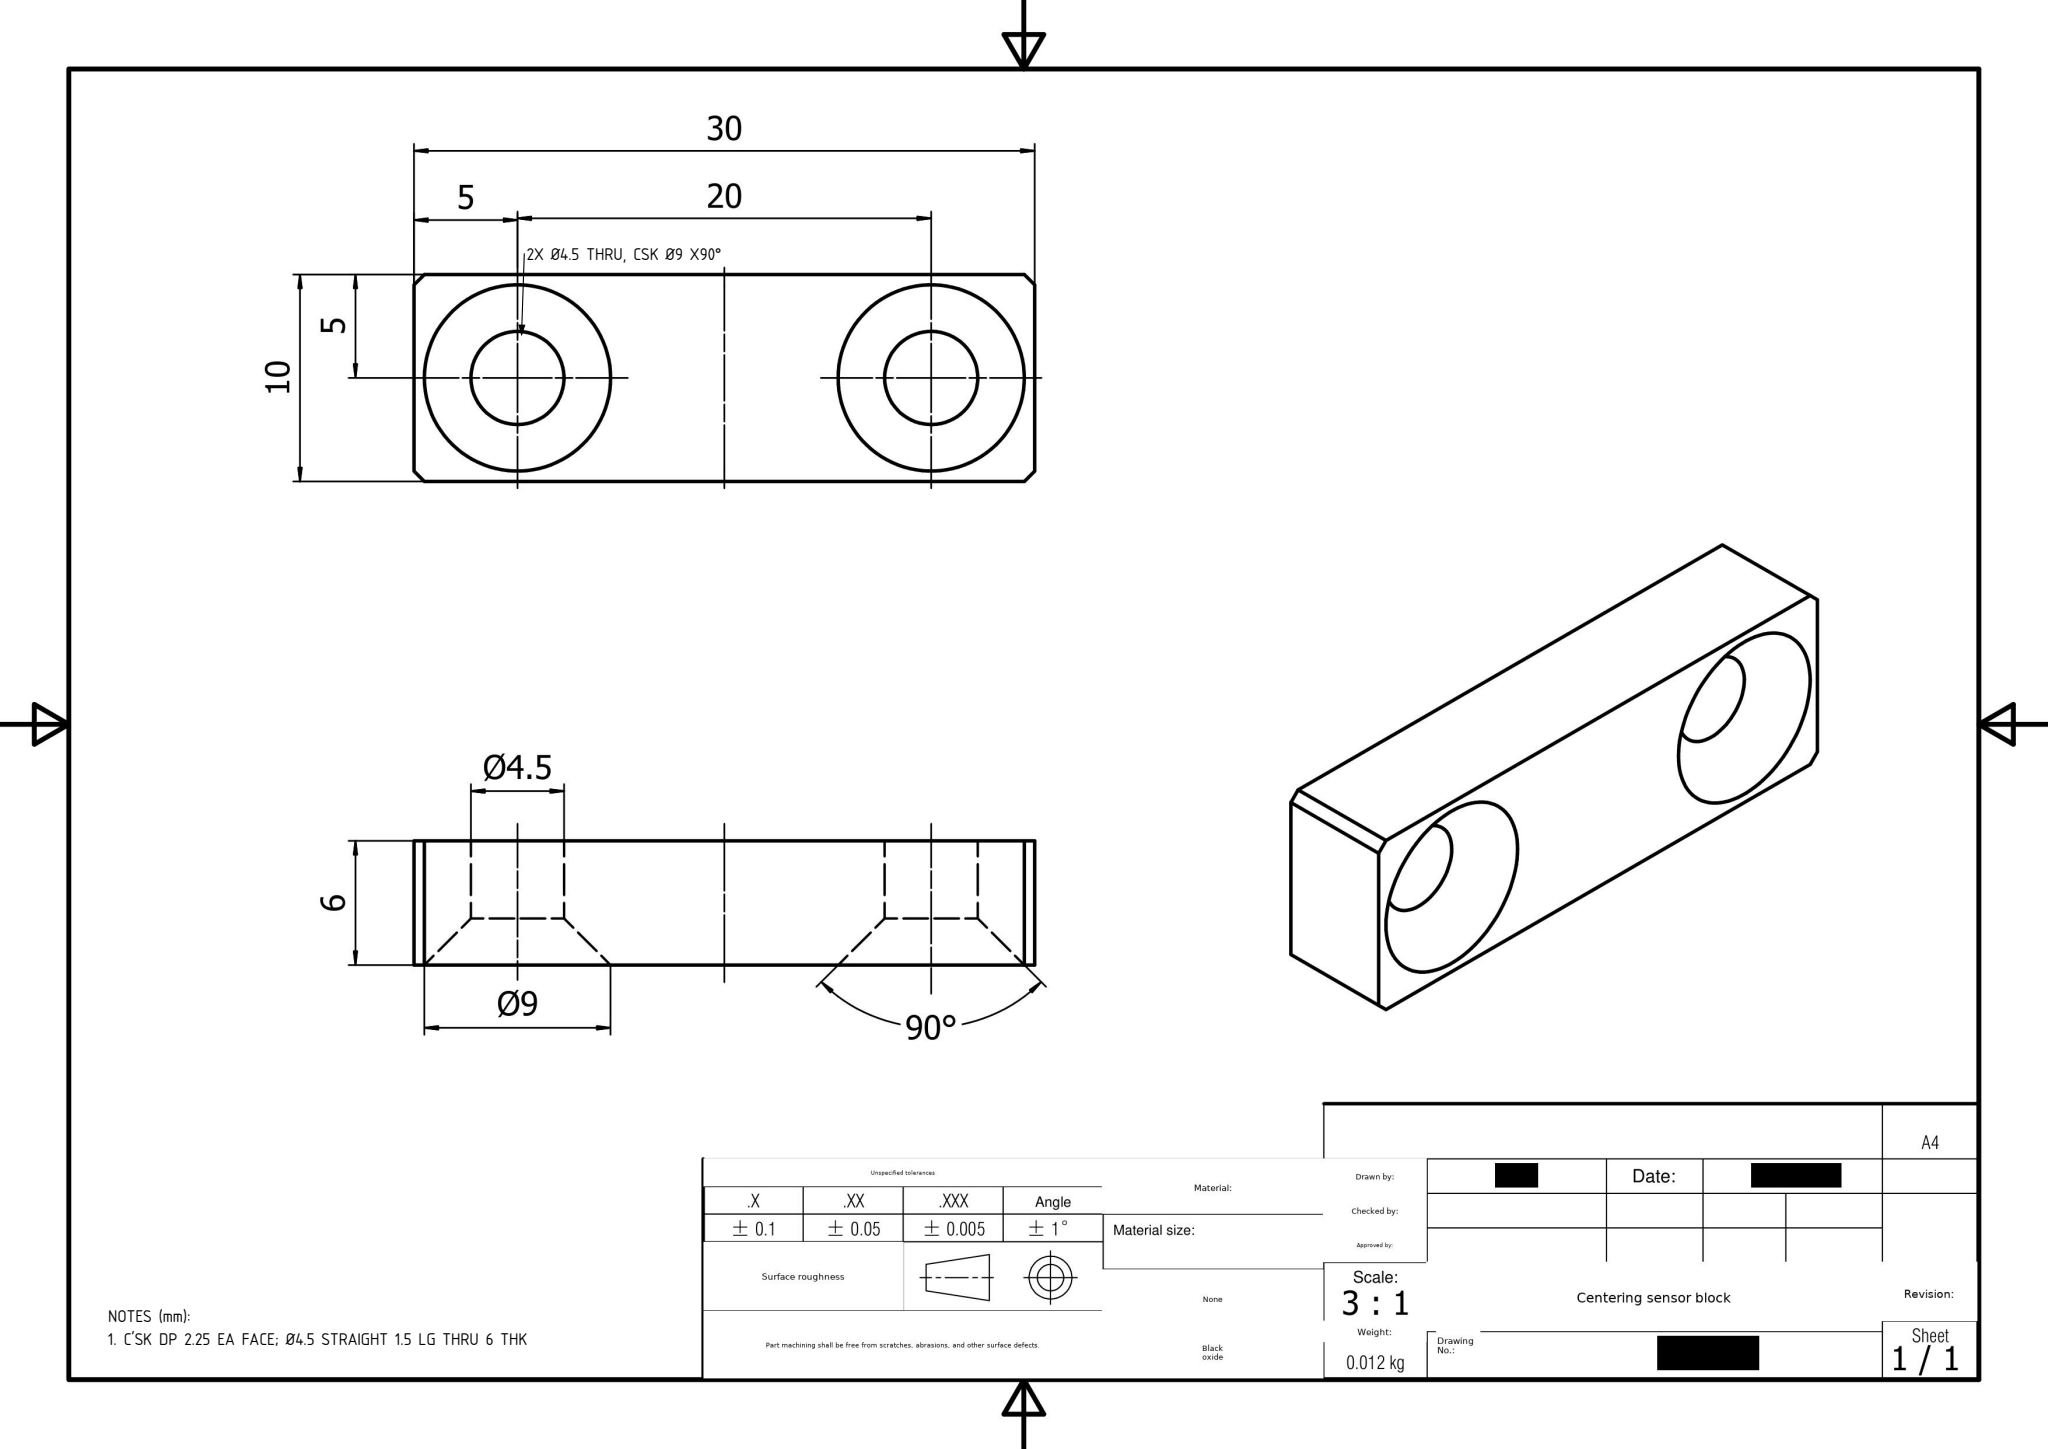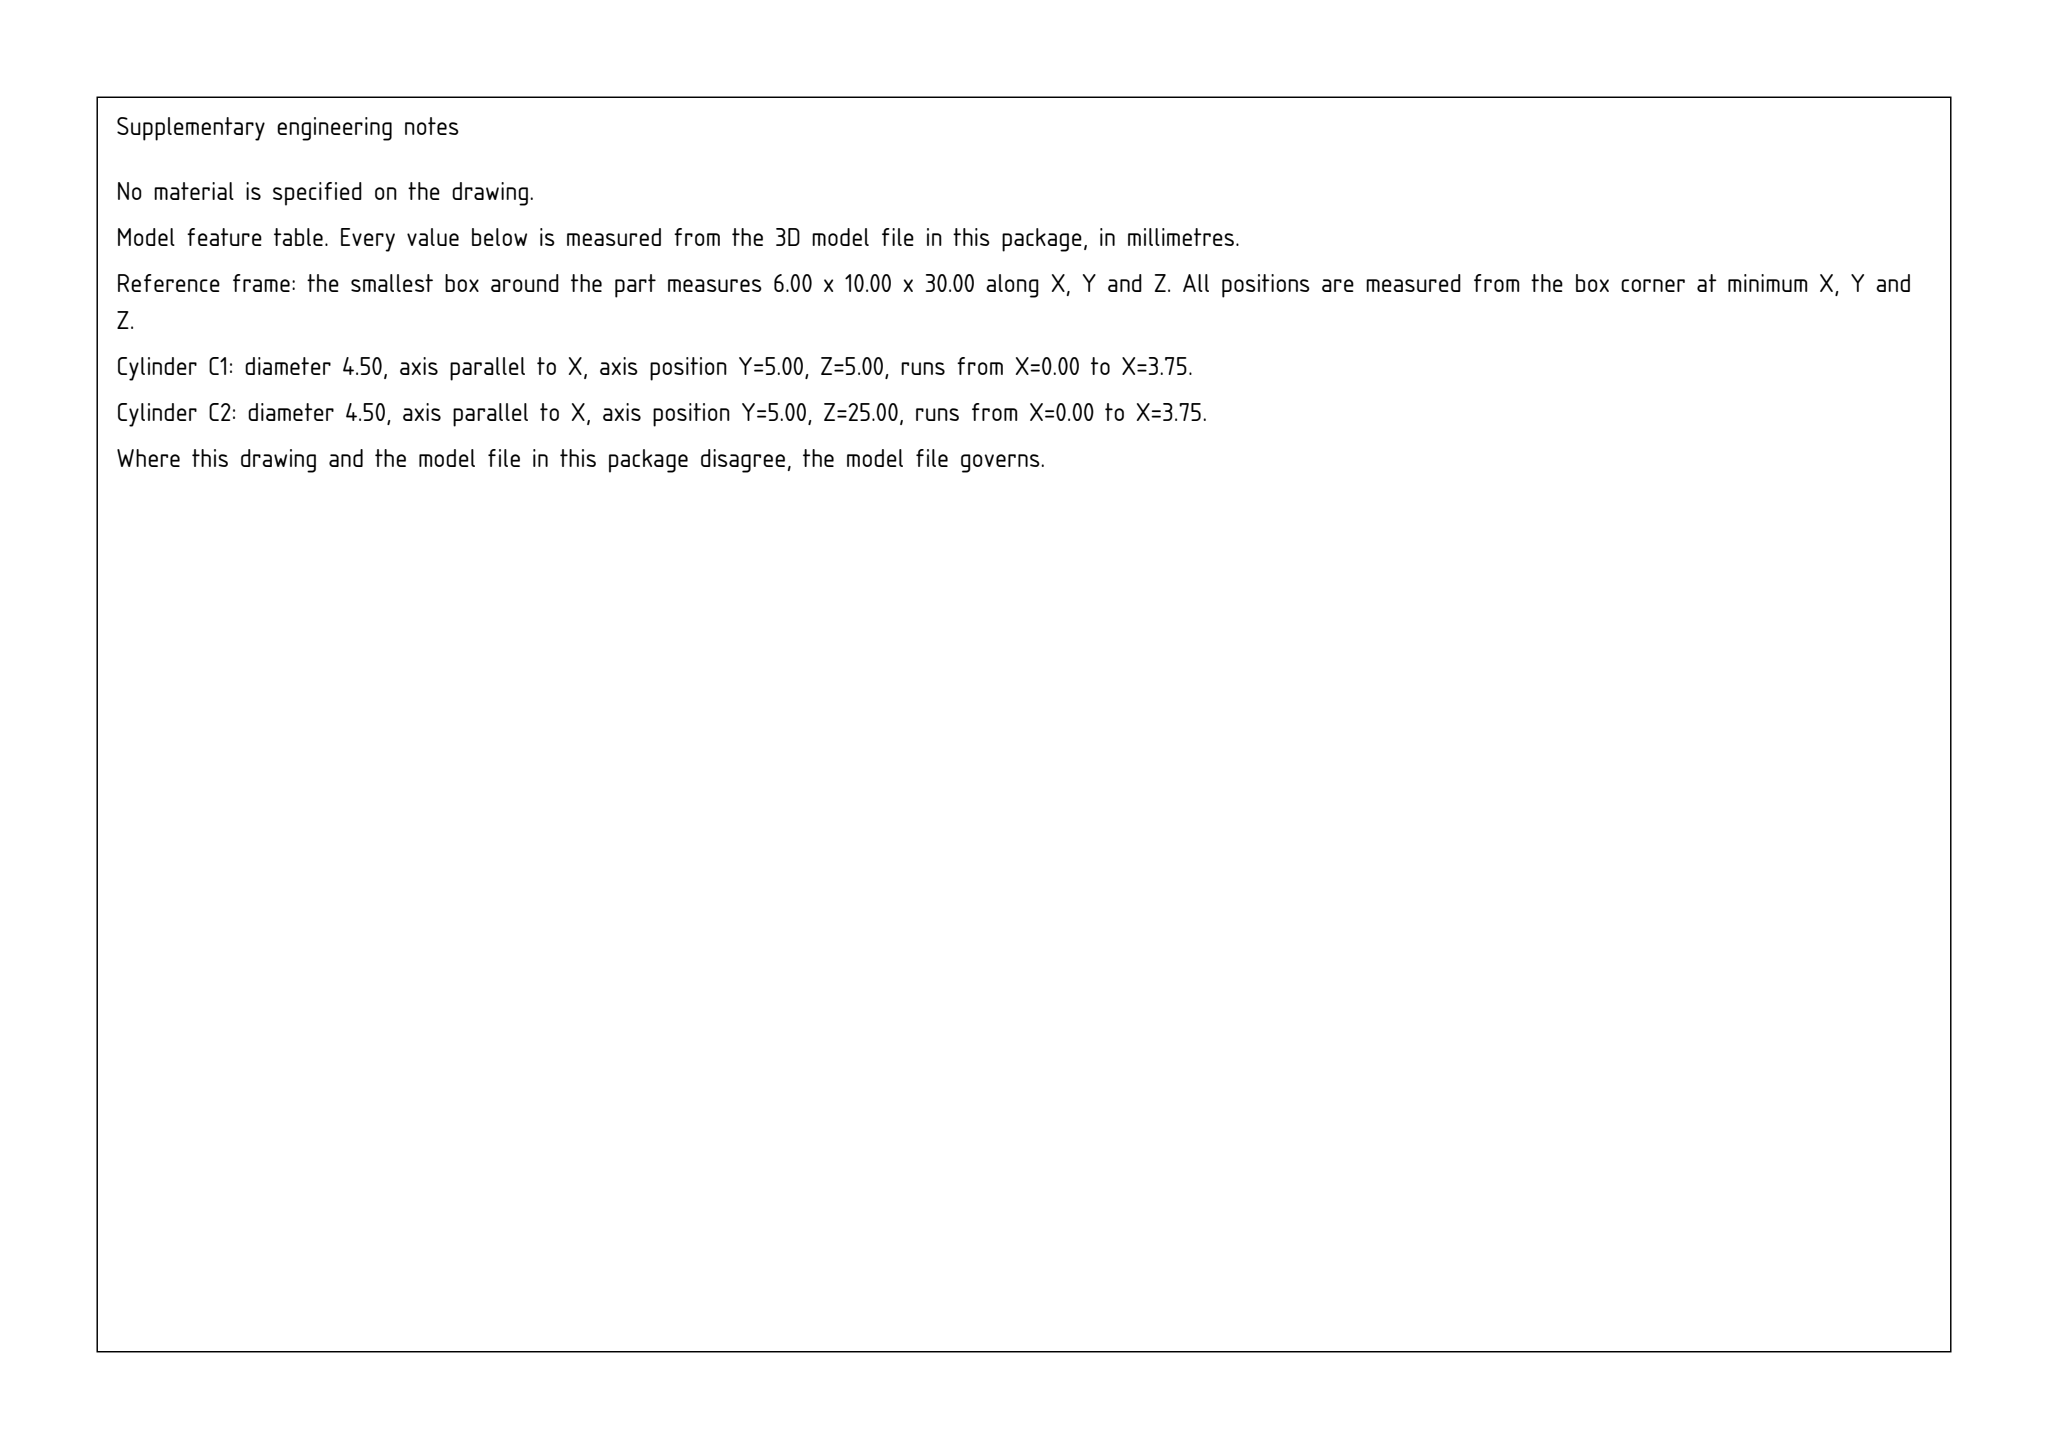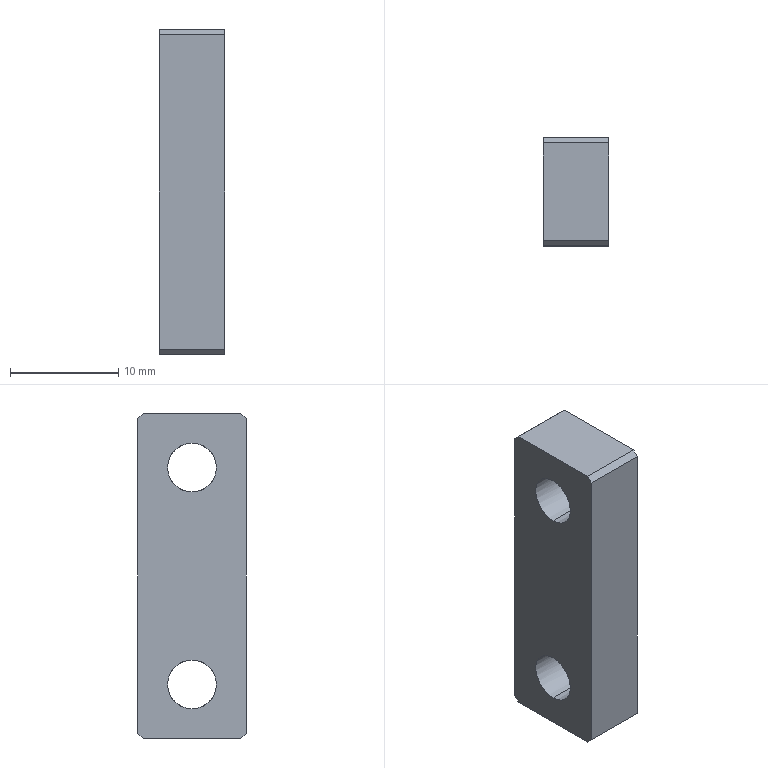Part | SolidWorks | mm | 1 solid | 18 faces | box 6 x 10 x 30 mm | volume 1511 mm3 | plane 10 | cylinder 4 | cone 4 | commonest cylinder face diameters 4.5 x4
Drawing notes:
Ø4.5 THRU, C'SK Ø9 X 90° BOTH FACES - 2 HOLES | from the solid: cylinders Ø4.5 axis x at (y5,z5)&(y5,z25), 2 per hole x 3.75 lg thru 6 thk; cones[90°,ref Ø9] qty 4 = 2 per hole
C'SK DP 2.25 EA FACE; Ø4.5 STRAIGHT 1.5 LG THRU 6 THK | from the solid: (9-4.5)/2=2.25 cone depth per face; bbox x=6, planes x=0 & x=6; 6-2(2.25)=1.5
STEP:
#1=CARTESIAN_POINT('',(0.,0.,-12.25));
#2=VERTEX_POINT('',#1);
#3=CARTESIAN_POINT('',(0.,0.,-7.75));
#4=VERTEX_POINT('',#3);
#5=CARTESIAN_POINT('',(0.,0.,-10.));
#6=DIRECTION('',(-1.,0.,0.));
#7=DIRECTION('',(0.,0.,-1.));
#8=AXIS2_PLACEMENT_3D('',#5,#6,#7);
#9=CIRCLE('',#8,2.25);
#10=EDGE_CURVE('',#2,#4,#9,.T.);
#11=ORIENTED_EDGE('',*,*,#10,.T.);
#12=CARTESIAN_POINT('',(3.75,0.,-7.75));
#13=VERTEX_POINT('',#12);
#14=CARTESIAN_POINT('',(-26.187,0.,-7.75));
#15=DIRECTION('',(1.,0.,0.));
#16=VECTOR('',#15,1000.);
#17=LINE('',#14,#16);
#18=EDGE_CURVE('',#4,#13,#17,.T.);
#19=ORIENTED_EDGE('',*,*,#18,.T.);
#20=CARTESIAN_POINT('',(3.75,-2.25,-10.));
#21=VERTEX_POINT('',#20);
#22=CARTESIAN_POINT('',(3.75,0.,-10.));
#23=DIRECTION('',(-1.,0.,0.));
#24=DIRECTION('',(0.,0.,-1.));
#25=AXIS2_PLACEMENT_3D('',#22,#23,#24);
#26=CIRCLE('',#25,2.25);
#27=EDGE_CURVE('',#21,#13,#26,.T.);
#28=ORIENTED_EDGE('',*,*,#27,.F.);
#29=CARTESIAN_POINT('',(3.75,0.,-12.25));
#30=VERTEX_POINT('',#29);
#31=CARTESIAN_POINT('',(3.75,0.,-10.));
#32=DIRECTION('',(-1.,0.,0.));
#33=DIRECTION('',(0.,0.,-1.));
#34=AXIS2_PLACEMENT_3D('',#31,#32,#33);
#35=CIRCLE('',#34,2.25);
#36=EDGE_CURVE('',#30,#21,#35,.T.);
#37=ORIENTED_EDGE('',*,*,#36,.F.);
#38=CARTESIAN_POINT('',(-26.187,0.,-12.25));
#39=DIRECTION('',(1.,0.,0.));
#40=VECTOR('',#39,1000.);
#41=LINE('',#38,#40);
#42=EDGE_CURVE('',#2,#30,#41,.T.);
#43=ORIENTED_EDGE('',*,*,#42,.F.);
#44=EDGE_LOOP('',(#11,#19,#28,#37,#43));
#45=FACE_OUTER_BOUND('',#44,.T.);
#46=CARTESIAN_POINT('',(-26.187,0.,-10.));
#47=DIRECTION('',(1.,0.,0.));
#48=DIRECTION('',(0.,0.,-1.));
#49=AXIS2_PLACEMENT_3D('',#46,#47,#48);
#50=CYLINDRICAL_SURFACE('',#49,2.25);
#51=ADVANCED_FACE('',(#45),#50,.F.);
#52=CARTESIAN_POINT('',(0.,0.,7.75));
#53=VERTEX_POINT('',#52);
#54=CARTESIAN_POINT('',(0.,0.,12.25));
#55=VERTEX_POINT('',#54);
#56=CARTESIAN_POINT('',(0.,0.,10.));
#57=DIRECTION('',(-1.,0.,0.));
#58=DIRECTION('',(0.,0.,-1.));
#59=AXIS2_PLACEMENT_3D('',#56,#57,#58);
#60=CIRCLE('',#59,2.25);
#61=EDGE_CURVE('',#53,#55,#60,.T.);
#62=ORIENTED_EDGE('',*,*,#61,.T.);
#63=CARTESIAN_POINT('',(3.75,0.,12.25));
#64=VERTEX_POINT('',#63);
#65=CARTESIAN_POINT('',(-26.187,0.,12.25));
#66=DIRECTION('',(1.,0.,0.));
#67=VECTOR('',#66,1000.);
#68=LINE('',#65,#67);
#69=EDGE_CURVE('',#55,#64,#68,.T.);
#70=ORIENTED_EDGE('',*,*,#69,.T.);
#71=CARTESIAN_POINT('',(3.75,-2.25,10.));
#72=VERTEX_POINT('',#71);
#73=CARTESIAN_POINT('',(3.75,0.,10.));
#74=DIRECTION('',(-1.,0.,0.));
#75=DIRECTION('',(0.,0.,-1.));
#76=AXIS2_PLACEMENT_3D('',#73,#74,#75);
#77=CIRCLE('',#76,2.25);
#78=EDGE_CURVE('',#72,#64,#77,.T.);
#79=ORIENTED_EDGE('',*,*,#78,.F.);
#80=CARTESIAN_POINT('',(3.75,0.,7.75));
#81=VERTEX_POINT('',#80);
#82=CARTESIAN_POINT('',(3.75,0.,10.));
#83=DIRECTION('',(-1.,0.,0.));
#84=DIRECTION('',(0.,0.,-1.));
#85=AXIS2_PLACEMENT_3D('',#82,#83,#84);
#86=CIRCLE('',#85,2.25);
#87=EDGE_CURVE('',#81,#72,#86,.T.);
#88=ORIENTED_EDGE('',*,*,#87,.F.);
#89=CARTESIAN_POINT('',(-26.187,0.,7.75));
#90=DIRECTION('',(1.,0.,0.));
#91=VECTOR('',#90,1000.);
#92=LINE('',#89,#91);
#93=EDGE_CURVE('',#53,#81,#92,.T.);
#94=ORIENTED_EDGE('',*,*,#93,.F.);
#95=EDGE_LOOP('',(#62,#70,#79,#88,#94));
#96=FACE_OUTER_BOUND('',#95,.T.);
#97=CARTESIAN_POINT('',(-26.187,0.,10.));
#98=DIRECTION('',(1.,0.,0.));
#99=DIRECTION('',(0.,0.,-1.));
#100=AXIS2_PLACEMENT_3D('',#97,#98,#99);
#101=CYLINDRICAL_SURFACE('',#100,2.25);
#102=ADVANCED_FACE('',(#96),#101,.F.);
#103=CARTESIAN_POINT('',(3.75,2.25,-10.));
#104=VERTEX_POINT('',#103);
#105=CARTESIAN_POINT('',(3.75,0.,-10.));
#106=DIRECTION('',(-1.,0.,0.));
#107=DIRECTION('',(0.,0.,-1.));
#108=AXIS2_PLACEMENT_3D('',#105,#106,#107);
#109=CIRCLE('',#108,2.25);
#110=EDGE_CURVE('',#104,#30,#109,.T.);
#111=ORIENTED_EDGE('',*,*,#110,.T.);
#112=ORIENTED_EDGE('',*,*,#36,.T.);
#113=CARTESIAN_POINT('',(6.,-4.5,-10.));
#114=VERTEX_POINT('',#113);
#115=CARTESIAN_POINT('',(6.,-4.5,-10.));
#116=DIRECTION('',(0.7071,-0.7071,0.));
#117=VECTOR('',#116,1000.);
#118=LINE('',#115,#117);
#119=EDGE_CURVE('',#21,#114,#118,.T.);
#120=ORIENTED_EDGE('',*,*,#119,.T.);
#121=CARTESIAN_POINT('',(6.,4.5,-10.));
#122=VERTEX_POINT('',#121);
#123=CARTESIAN_POINT('',(6.,0.,-10.));
#124=DIRECTION('',(-1.,-0.,0.));
#125=DIRECTION('',(-0.,1.,0.));
#126=AXIS2_PLACEMENT_3D('',#123,#124,#125);
#127=CIRCLE('',#126,4.5);
#128=EDGE_CURVE('',#122,#114,#127,.T.);
#129=ORIENTED_EDGE('',*,*,#128,.F.);
#130=CARTESIAN_POINT('',(6.,4.5,-10.));
#131=DIRECTION('',(0.7071,0.7071,0.));
#132=VECTOR('',#131,1000.);
#133=LINE('',#130,#132);
#134=EDGE_CURVE('',#104,#122,#133,.T.);
#135=ORIENTED_EDGE('',*,*,#134,.F.);
#136=EDGE_LOOP('',(#111,#112,#120,#129,#135));
#137=FACE_OUTER_BOUND('',#136,.T.);
#138=CARTESIAN_POINT('',(6.,0.,-10.));
#139=DIRECTION('',(1.,0.,0.));
#140=DIRECTION('',(-0.,1.,0.));
#141=AXIS2_PLACEMENT_3D('',#138,#139,#140);
#142=CONICAL_SURFACE('',#141,4.5,0.7854);
#143=ADVANCED_FACE('',(#137),#142,.F.);
#144=CARTESIAN_POINT('',(3.75,2.25,10.));
#145=VERTEX_POINT('',#144);
#146=CARTESIAN_POINT('',(3.75,0.,10.));
#147=DIRECTION('',(-1.,0.,0.));
#148=DIRECTION('',(0.,0.,-1.));
#149=AXIS2_PLACEMENT_3D('',#146,#147,#148);
#150=CIRCLE('',#149,2.25);
#151=EDGE_CURVE('',#145,#81,#150,.T.);
#152=ORIENTED_EDGE('',*,*,#151,.T.);
#153=ORIENTED_EDGE('',*,*,#87,.T.);
#154=CARTESIAN_POINT('',(6.,-4.5,10.));
#155=VERTEX_POINT('',#154);
#156=CARTESIAN_POINT('',(6.,-4.5,10.));
#157=DIRECTION('',(0.7071,-0.7071,0.));
#158=VECTOR('',#157,1000.);
#159=LINE('',#156,#158);
#160=EDGE_CURVE('',#72,#155,#159,.T.);
#161=ORIENTED_EDGE('',*,*,#160,.T.);
#162=CARTESIAN_POINT('',(6.,4.5,10.));
#163=VERTEX_POINT('',#162);
#164=CARTESIAN_POINT('',(6.,0.,10.));
#165=DIRECTION('',(-1.,-0.,0.));
#166=DIRECTION('',(-0.,1.,0.));
#167=AXIS2_PLACEMENT_3D('',#164,#165,#166);
#168=CIRCLE('',#167,4.5);
#169=EDGE_CURVE('',#163,#155,#168,.T.);
#170=ORIENTED_EDGE('',*,*,#169,.F.);
#171=CARTESIAN_POINT('',(6.,4.5,10.));
#172=DIRECTION('',(0.7071,0.7071,0.));
#173=VECTOR('',#172,1000.);
#174=LINE('',#171,#173);
#175=EDGE_CURVE('',#145,#163,#174,.T.);
#176=ORIENTED_EDGE('',*,*,#175,.F.);
#177=EDGE_LOOP('',(#152,#153,#161,#170,#176));
#178=FACE_OUTER_BOUND('',#177,.T.);
#179=CARTESIAN_POINT('',(6.,0.,10.));
#180=DIRECTION('',(1.,0.,0.));
#181=DIRECTION('',(0.,1.,0.));
#182=AXIS2_PLACEMENT_3D('',#179,#180,#181);
#183=CONICAL_SURFACE('',#182,4.5,0.7854);
#184=ADVANCED_FACE('',(#178),#183,.F.);
#185=ORIENTED_EDGE('',*,*,#10,.F.);
#186=CARTESIAN_POINT('',(0.,0.,-10.));
#187=DIRECTION('',(-1.,0.,0.));
#188=DIRECTION('',(0.,0.,-1.));
#189=AXIS2_PLACEMENT_3D('',#186,#187,#188);
#190=CIRCLE('',#189,2.25);
#191=EDGE_CURVE('',#4,#2,#190,.T.);
#192=ORIENTED_EDGE('',*,*,#191,.F.);
#193=EDGE_LOOP('',(#185,#192));
#194=FACE_BOUND('',#193,.T.);
#195=ORIENTED_EDGE('',*,*,#61,.F.);
#196=CARTESIAN_POINT('',(0.,0.,10.));
#197=DIRECTION('',(-1.,0.,0.));
#198=DIRECTION('',(0.,0.,-1.));
#199=AXIS2_PLACEMENT_3D('',#196,#197,#198);
#200=CIRCLE('',#199,2.25);
#201=EDGE_CURVE('',#55,#53,#200,.T.);
#202=ORIENTED_EDGE('',*,*,#201,.F.);
#203=EDGE_LOOP('',(#195,#202));
#204=FACE_BOUND('',#203,.T.);
#205=CARTESIAN_POINT('',(0.,-5.,14.5));
#206=VERTEX_POINT('',#205);
#207=CARTESIAN_POINT('',(0.,-5.,-14.5));
#208=VERTEX_POINT('',#207);
#209=CARTESIAN_POINT('',(0.,-5.,0.));
#210=DIRECTION('',(0.,0.,-1.));
#211=VECTOR('',#210,1000.);
#212=LINE('',#209,#211);
#213=EDGE_CURVE('',#206,#208,#212,.T.);
#214=ORIENTED_EDGE('',*,*,#213,.F.);
#215=CARTESIAN_POINT('',(0.,-4.5,15.));
#216=VERTEX_POINT('',#215);
#217=CARTESIAN_POINT('',(0.,-4.75,14.75));
#218=DIRECTION('',(0.,-0.7071,-0.7071));
#219=VECTOR('',#218,1000.);
#220=LINE('',#217,#219);
#221=EDGE_CURVE('',#216,#206,#220,.T.);
#222=ORIENTED_EDGE('',*,*,#221,.F.);
#223=CARTESIAN_POINT('',(0.,4.5,15.));
#224=VERTEX_POINT('',#223);
#225=CARTESIAN_POINT('',(0.,0.,15.));
#226=DIRECTION('',(0.,-1.,0.));
#227=VECTOR('',#226,1000.);
#228=LINE('',#225,#227);
#229=EDGE_CURVE('',#224,#216,#228,.T.);
#230=ORIENTED_EDGE('',*,*,#229,.F.);
#231=CARTESIAN_POINT('',(0.,5.,14.5));
#232=VERTEX_POINT('',#231);
#233=CARTESIAN_POINT('',(0.,4.75,14.75));
#234=DIRECTION('',(0.,-0.7071,0.7071));
#235=VECTOR('',#234,1000.);
#236=LINE('',#233,#235);
#237=EDGE_CURVE('',#232,#224,#236,.T.);
#238=ORIENTED_EDGE('',*,*,#237,.F.);
#239=CARTESIAN_POINT('',(0.,5.,-14.5));
#240=VERTEX_POINT('',#239);
#241=CARTESIAN_POINT('',(0.,5.,0.));
#242=DIRECTION('',(0.,0.,1.));
#243=VECTOR('',#242,1000.);
#244=LINE('',#241,#243);
#245=EDGE_CURVE('',#240,#232,#244,.T.);
#246=ORIENTED_EDGE('',*,*,#245,.F.);
#247=CARTESIAN_POINT('',(0.,4.5,-15.));
#248=VERTEX_POINT('',#247);
#249=CARTESIAN_POINT('',(0.,4.75,-14.75));
#250=DIRECTION('',(0.,0.7071,0.7071));
#251=VECTOR('',#250,1000.);
#252=LINE('',#249,#251);
#253=EDGE_CURVE('',#248,#240,#252,.T.);
#254=ORIENTED_EDGE('',*,*,#253,.F.);
#255=CARTESIAN_POINT('',(0.,-4.5,-15.));
#256=VERTEX_POINT('',#255);
#257=CARTESIAN_POINT('',(0.,0.,-15.));
#258=DIRECTION('',(0.,1.,0.));
#259=VECTOR('',#258,1000.);
#260=LINE('',#257,#259);
#261=EDGE_CURVE('',#256,#248,#260,.T.);
#262=ORIENTED_EDGE('',*,*,#261,.F.);
#263=CARTESIAN_POINT('',(0.,-4.75,-14.75));
#264=DIRECTION('',(0.,0.7071,-0.7071));
#265=VECTOR('',#264,1000.);
#266=LINE('',#263,#265);
#267=EDGE_CURVE('',#208,#256,#266,.T.);
#268=ORIENTED_EDGE('',*,*,#267,.F.);
#269=EDGE_LOOP('',(#214,#222,#230,#238,#246,#254,#262,#268));
#270=FACE_OUTER_BOUND('',#269,.T.);
#271=CARTESIAN_POINT('',(0.,0.,0.));
#272=DIRECTION('',(1.,0.,0.));
#273=DIRECTION('',(0.,0.,-1.));
#274=AXIS2_PLACEMENT_3D('',#271,#272,#273);
#275=PLANE('',#274);
#276=ADVANCED_FACE('',(#194,#204,#270),#275,.F.);
#277=ORIENTED_EDGE('',*,*,#18,.F.);
#278=ORIENTED_EDGE('',*,*,#191,.T.);
#279=ORIENTED_EDGE('',*,*,#42,.T.);
#280=ORIENTED_EDGE('',*,*,#110,.F.);
#281=CARTESIAN_POINT('',(3.75,0.,-10.));
#282=DIRECTION('',(-1.,0.,0.));
#283=DIRECTION('',(0.,0.,-1.));
#284=AXIS2_PLACEMENT_3D('',#281,#282,#283);
#285=CIRCLE('',#284,2.25);
#286=EDGE_CURVE('',#13,#104,#285,.T.);
#287=ORIENTED_EDGE('',*,*,#286,.F.);
#288=EDGE_LOOP('',(#277,#278,#279,#280,#287));
#289=FACE_OUTER_BOUND('',#288,.T.);
#290=CARTESIAN_POINT('',(-26.187,0.,-10.));
#291=DIRECTION('',(1.,0.,0.));
#292=DIRECTION('',(0.,0.,-1.));
#293=AXIS2_PLACEMENT_3D('',#290,#291,#292);
#294=CYLINDRICAL_SURFACE('',#293,2.25);
#295=ADVANCED_FACE('',(#289),#294,.F.);
#296=ORIENTED_EDGE('',*,*,#69,.F.);
#297=ORIENTED_EDGE('',*,*,#201,.T.);
#298=ORIENTED_EDGE('',*,*,#93,.T.);
#299=ORIENTED_EDGE('',*,*,#151,.F.);
#300=CARTESIAN_POINT('',(3.75,0.,10.));
#301=DIRECTION('',(-1.,0.,0.));
#302=DIRECTION('',(0.,0.,-1.));
#303=AXIS2_PLACEMENT_3D('',#300,#301,#302);
#304=CIRCLE('',#303,2.25);
#305=EDGE_CURVE('',#64,#145,#304,.T.);
#306=ORIENTED_EDGE('',*,*,#305,.F.);
#307=EDGE_LOOP('',(#296,#297,#298,#299,#306));
#308=FACE_OUTER_BOUND('',#307,.T.);
#309=CARTESIAN_POINT('',(-26.187,0.,10.));
#310=DIRECTION('',(1.,0.,0.));
#311=DIRECTION('',(0.,0.,-1.));
#312=AXIS2_PLACEMENT_3D('',#309,#310,#311);
#313=CYLINDRICAL_SURFACE('',#312,2.25);
#314=ADVANCED_FACE('',(#308),#313,.F.);
#315=CARTESIAN_POINT('',(6.,-5.,14.5));
#316=VERTEX_POINT('',#315);
#317=CARTESIAN_POINT('',(0.,-5.,14.5));
#318=DIRECTION('',(-1.,0.,0.));
#319=VECTOR('',#318,1000.);
#320=LINE('',#317,#319);
#321=EDGE_CURVE('',#316,#206,#320,.T.);
#322=ORIENTED_EDGE('',*,*,#321,.T.);
#323=ORIENTED_EDGE('',*,*,#213,.T.);
#324=CARTESIAN_POINT('',(6.,-5.,-14.5));
#325=VERTEX_POINT('',#324);
#326=CARTESIAN_POINT('',(0.,-5.,-14.5));
#327=DIRECTION('',(1.,0.,0.));
#328=VECTOR('',#327,1000.);
#329=LINE('',#326,#328);
#330=EDGE_CURVE('',#208,#325,#329,.T.);
#331=ORIENTED_EDGE('',*,*,#330,.T.);
#332=CARTESIAN_POINT('',(6.,-5.,15.));
#333=DIRECTION('',(0.,0.,1.));
#334=VECTOR('',#333,1000.);
#335=LINE('',#332,#334);
#336=EDGE_CURVE('',#325,#316,#335,.T.);
#337=ORIENTED_EDGE('',*,*,#336,.T.);
#338=EDGE_LOOP('',(#322,#323,#331,#337));
#339=FACE_OUTER_BOUND('',#338,.T.);
#340=CARTESIAN_POINT('',(0.,-5.,15.));
#341=DIRECTION('',(0.,-1.,0.));
#342=DIRECTION('',(0.,0.,-1.));
#343=AXIS2_PLACEMENT_3D('',#340,#341,#342);
#344=PLANE('',#343);
#345=ADVANCED_FACE('',(#339),#344,.T.);
#346=CARTESIAN_POINT('',(6.,-4.5,15.));
#347=VERTEX_POINT('',#346);
#348=CARTESIAN_POINT('',(0.,-4.5,15.));
#349=DIRECTION('',(1.,0.,0.));
#350=VECTOR('',#349,1000.);
#351=LINE('',#348,#350);
#352=EDGE_CURVE('',#216,#347,#351,.T.);
#353=ORIENTED_EDGE('',*,*,#352,.T.);
#354=CARTESIAN_POINT('',(6.,4.5,15.));
#355=VERTEX_POINT('',#354);
#356=CARTESIAN_POINT('',(6.,5.,15.));
#357=DIRECTION('',(0.,1.,0.));
#358=VECTOR('',#357,1000.);
#359=LINE('',#356,#358);
#360=EDGE_CURVE('',#347,#355,#359,.T.);
#361=ORIENTED_EDGE('',*,*,#360,.T.);
#362=CARTESIAN_POINT('',(0.,4.5,15.));
#363=DIRECTION('',(-1.,0.,0.));
#364=VECTOR('',#363,1000.);
#365=LINE('',#362,#364);
#366=EDGE_CURVE('',#355,#224,#365,.T.);
#367=ORIENTED_EDGE('',*,*,#366,.T.);
#368=ORIENTED_EDGE('',*,*,#229,.T.);
#369=EDGE_LOOP('',(#353,#361,#367,#368));
#370=FACE_OUTER_BOUND('',#369,.T.);
#371=CARTESIAN_POINT('',(0.,5.,15.));
#372=DIRECTION('',(0.,0.,1.));
#373=DIRECTION('',(1.,0.,0.));
#374=AXIS2_PLACEMENT_3D('',#371,#372,#373);
#375=PLANE('',#374);
#376=ADVANCED_FACE('',(#370),#375,.T.);
#377=CARTESIAN_POINT('',(6.,5.,14.5));
#378=VERTEX_POINT('',#377);
#379=CARTESIAN_POINT('',(0.,5.,14.5));
#380=DIRECTION('',(1.,0.,0.));
#381=VECTOR('',#380,1000.);
#382=LINE('',#379,#381);
#383=EDGE_CURVE('',#232,#378,#382,.T.);
#384=ORIENTED_EDGE('',*,*,#383,.T.);
#385=CARTESIAN_POINT('',(6.,5.,-14.5));
#386=VERTEX_POINT('',#385);
#387=CARTESIAN_POINT('',(6.,5.,-15.));
#388=DIRECTION('',(0.,0.,-1.));
#389=VECTOR('',#388,1000.);
#390=LINE('',#387,#389);
#391=EDGE_CURVE('',#378,#386,#390,.T.);
#392=ORIENTED_EDGE('',*,*,#391,.T.);
#393=CARTESIAN_POINT('',(0.,5.,-14.5));
#394=DIRECTION('',(-1.,0.,0.));
#395=VECTOR('',#394,1000.);
#396=LINE('',#393,#395);
#397=EDGE_CURVE('',#386,#240,#396,.T.);
#398=ORIENTED_EDGE('',*,*,#397,.T.);
#399=ORIENTED_EDGE('',*,*,#245,.T.);
#400=EDGE_LOOP('',(#384,#392,#398,#399));
#401=FACE_OUTER_BOUND('',#400,.T.);
#402=CARTESIAN_POINT('',(0.,5.,-15.));
#403=DIRECTION('',(0.,1.,0.));
#404=DIRECTION('',(0.,0.,1.));
#405=AXIS2_PLACEMENT_3D('',#402,#403,#404);
#406=PLANE('',#405);
#407=ADVANCED_FACE('',(#401),#406,.T.);
#408=CARTESIAN_POINT('',(6.,4.5,-15.));
#409=VERTEX_POINT('',#408);
#410=CARTESIAN_POINT('',(0.,4.5,-15.));
#411=DIRECTION('',(1.,0.,0.));
#412=VECTOR('',#411,1000.);
#413=LINE('',#410,#412);
#414=EDGE_CURVE('',#248,#409,#413,.T.);
#415=ORIENTED_EDGE('',*,*,#414,.T.);
#416=CARTESIAN_POINT('',(6.,-4.5,-15.));
#417=VERTEX_POINT('',#416);
#418=CARTESIAN_POINT('',(6.,-5.,-15.));
#419=DIRECTION('',(0.,-1.,0.));
#420=VECTOR('',#419,1000.);
#421=LINE('',#418,#420);
#422=EDGE_CURVE('',#409,#417,#421,.T.);
#423=ORIENTED_EDGE('',*,*,#422,.T.);
#424=CARTESIAN_POINT('',(0.,-4.5,-15.));
#425=DIRECTION('',(-1.,0.,0.));
#426=VECTOR('',#425,1000.);
#427=LINE('',#424,#426);
#428=EDGE_CURVE('',#417,#256,#427,.T.);
#429=ORIENTED_EDGE('',*,*,#428,.T.);
#430=ORIENTED_EDGE('',*,*,#261,.T.);
#431=EDGE_LOOP('',(#415,#423,#429,#430));
#432=FACE_OUTER_BOUND('',#431,.T.);
#433=CARTESIAN_POINT('',(0.,-5.,-15.));
#434=DIRECTION('',(0.,0.,-1.));
#435=DIRECTION('',(-1.,0.,0.));
#436=AXIS2_PLACEMENT_3D('',#433,#434,#435);
#437=PLANE('',#436);
#438=ADVANCED_FACE('',(#432),#437,.T.);
#439=ORIENTED_EDGE('',*,*,#119,.F.);
#440=ORIENTED_EDGE('',*,*,#27,.T.);
#441=ORIENTED_EDGE('',*,*,#286,.T.);
#442=ORIENTED_EDGE('',*,*,#134,.T.);
#443=CARTESIAN_POINT('',(6.,0.,-10.));
#444=DIRECTION('',(-1.,-0.,0.));
#445=DIRECTION('',(-0.,1.,0.));
#446=AXIS2_PLACEMENT_3D('',#443,#444,#445);
#447=CIRCLE('',#446,4.5);
#448=EDGE_CURVE('',#114,#122,#447,.T.);
#449=ORIENTED_EDGE('',*,*,#448,.F.);
#450=EDGE_LOOP('',(#439,#440,#441,#442,#449));
#451=FACE_OUTER_BOUND('',#450,.T.);
#452=CARTESIAN_POINT('',(6.,0.,-10.));
#453=DIRECTION('',(1.,0.,0.));
#454=DIRECTION('',(-0.,1.,0.));
#455=AXIS2_PLACEMENT_3D('',#452,#453,#454);
#456=CONICAL_SURFACE('',#455,4.5,0.7854);
#457=ADVANCED_FACE('',(#451),#456,.F.);
#458=ORIENTED_EDGE('',*,*,#160,.F.);
#459=ORIENTED_EDGE('',*,*,#78,.T.);
#460=ORIENTED_EDGE('',*,*,#305,.T.);
#461=ORIENTED_EDGE('',*,*,#175,.T.);
#462=CARTESIAN_POINT('',(6.,0.,10.));
#463=DIRECTION('',(-1.,-0.,0.));
#464=DIRECTION('',(-0.,1.,0.));
#465=AXIS2_PLACEMENT_3D('',#462,#463,#464);
#466=CIRCLE('',#465,4.5);
#467=EDGE_CURVE('',#155,#163,#466,.T.);
#468=ORIENTED_EDGE('',*,*,#467,.F.);
#469=EDGE_LOOP('',(#458,#459,#460,#461,#468));
#470=FACE_OUTER_BOUND('',#469,.T.);
#471=CARTESIAN_POINT('',(6.,0.,10.));
#472=DIRECTION('',(1.,0.,0.));
#473=DIRECTION('',(0.,1.,0.));
#474=AXIS2_PLACEMENT_3D('',#471,#472,#473);
#475=CONICAL_SURFACE('',#474,4.5,0.7854);
#476=ADVANCED_FACE('',(#470),#475,.F.);
#477=ORIENTED_EDGE('',*,*,#221,.T.);
#478=ORIENTED_EDGE('',*,*,#321,.F.);
#479=CARTESIAN_POINT('',(6.,-4.75,14.75));
#480=DIRECTION('',(0.,0.7071,0.7071));
#481=VECTOR('',#480,1000.);
#482=LINE('',#479,#481);
#483=EDGE_CURVE('',#316,#347,#482,.T.);
#484=ORIENTED_EDGE('',*,*,#483,.T.);
#485=ORIENTED_EDGE('',*,*,#352,.F.);
#486=EDGE_LOOP('',(#477,#478,#484,#485));
#487=FACE_OUTER_BOUND('',#486,.T.);
#488=CARTESIAN_POINT('',(0.,-4.75,14.75));
#489=DIRECTION('',(0.,-0.7071,0.7071));
#490=DIRECTION('',(0.,-0.7071,-0.7071));
#491=AXIS2_PLACEMENT_3D('',#488,#489,#490);
#492=PLANE('',#491);
#493=ADVANCED_FACE('',(#487),#492,.T.);
#494=ORIENTED_EDGE('',*,*,#128,.T.);
#495=ORIENTED_EDGE('',*,*,#448,.T.);
#496=EDGE_LOOP('',(#494,#495));
#497=FACE_BOUND('',#496,.T.);
#498=ORIENTED_EDGE('',*,*,#169,.T.);
#499=ORIENTED_EDGE('',*,*,#467,.T.);
#500=EDGE_LOOP('',(#498,#499));
#501=FACE_BOUND('',#500,.T.);
#502=ORIENTED_EDGE('',*,*,#483,.F.);
#503=ORIENTED_EDGE('',*,*,#336,.F.);
#504=CARTESIAN_POINT('',(6.,-5.,-14.5));
#505=DIRECTION('',(0.,0.7071,-0.7071));
#506=VECTOR('',#505,1000.);
#507=LINE('',#504,#506);
#508=EDGE_CURVE('',#325,#417,#507,.T.);
#509=ORIENTED_EDGE('',*,*,#508,.T.);
#510=ORIENTED_EDGE('',*,*,#422,.F.);
#511=CARTESIAN_POINT('',(6.,4.5,-15.));
#512=DIRECTION('',(0.,0.7071,0.7071));
#513=VECTOR('',#512,1000.);
#514=LINE('',#511,#513);
#515=EDGE_CURVE('',#409,#386,#514,.T.);
#516=ORIENTED_EDGE('',*,*,#515,.T.);
#517=ORIENTED_EDGE('',*,*,#391,.F.);
#518=CARTESIAN_POINT('',(6.,5.,14.5));
#519=DIRECTION('',(0.,-0.7071,0.7071));
#520=VECTOR('',#519,1000.);
#521=LINE('',#518,#520);
#522=EDGE_CURVE('',#378,#355,#521,.T.);
#523=ORIENTED_EDGE('',*,*,#522,.T.);
#524=ORIENTED_EDGE('',*,*,#360,.F.);
#525=EDGE_LOOP('',(#502,#503,#509,#510,#516,#517,#523,#524));
#526=FACE_OUTER_BOUND('',#525,.T.);
#527=CARTESIAN_POINT('',(6.,0.,0.));
#528=DIRECTION('',(1.,0.,0.));
#529=DIRECTION('',(0.,0.,-1.));
#530=AXIS2_PLACEMENT_3D('',#527,#528,#529);
#531=PLANE('',#530);
#532=ADVANCED_FACE('',(#497,#501,#526),#531,.T.);
#533=ORIENTED_EDGE('',*,*,#267,.T.);
#534=ORIENTED_EDGE('',*,*,#428,.F.);
#535=ORIENTED_EDGE('',*,*,#508,.F.);
#536=ORIENTED_EDGE('',*,*,#330,.F.);
#537=EDGE_LOOP('',(#533,#534,#535,#536));
#538=FACE_OUTER_BOUND('',#537,.T.);
#539=CARTESIAN_POINT('',(0.,-4.75,-14.75));
#540=DIRECTION('',(0.,-0.7071,-0.7071));
#541=DIRECTION('',(0.,0.7071,-0.7071));
#542=AXIS2_PLACEMENT_3D('',#539,#540,#541);
#543=PLANE('',#542);
#544=ADVANCED_FACE('',(#538),#543,.T.);
#545=ORIENTED_EDGE('',*,*,#237,.T.);
#546=ORIENTED_EDGE('',*,*,#366,.F.);
#547=ORIENTED_EDGE('',*,*,#522,.F.);
#548=ORIENTED_EDGE('',*,*,#383,.F.);
#549=EDGE_LOOP('',(#545,#546,#547,#548));
#550=FACE_OUTER_BOUND('',#549,.T.);
#551=CARTESIAN_POINT('',(0.,4.75,14.75));
#552=DIRECTION('',(0.,0.7071,0.7071));
#553=DIRECTION('',(0.,-0.7071,0.7071));
#554=AXIS2_PLACEMENT_3D('',#551,#552,#553);
#555=PLANE('',#554);
#556=ADVANCED_FACE('',(#550),#555,.T.);
#557=ORIENTED_EDGE('',*,*,#253,.T.);
#558=ORIENTED_EDGE('',*,*,#397,.F.);
#559=ORIENTED_EDGE('',*,*,#515,.F.);
#560=ORIENTED_EDGE('',*,*,#414,.F.);
#561=EDGE_LOOP('',(#557,#558,#559,#560));
#562=FACE_OUTER_BOUND('',#561,.T.);
#563=CARTESIAN_POINT('',(0.,4.75,-14.75));
#564=DIRECTION('',(0.,0.7071,-0.7071));
#565=DIRECTION('',(0.,0.7071,0.7071));
#566=AXIS2_PLACEMENT_3D('',#563,#564,#565);
#567=PLANE('',#566);
#568=ADVANCED_FACE('',(#562),#567,.T.);
#569=CLOSED_SHELL('',(#51,#102,#143,#184,#276,#295,#314,#345,#376,#407,#438,#457,#476,#493,#532,#544,#556,#568));
#570=MANIFOLD_SOLID_BREP('',#569);
#571=CARTESIAN_POINT('',(0.,0.,0.));
#572=DIRECTION('',(0.,0.,1.));
#573=DIRECTION('',(1.,0.,0.));
#574=AXIS2_PLACEMENT_3D('',#571,#572,#573);
#575=(LENGTH_UNIT()NAMED_UNIT(*)SI_UNIT(.MILLI.,.METRE.));
#576=UNCERTAINTY_MEASURE_WITH_UNIT(LENGTH_MEASURE(0.00001),#575,'','');
#577=(NAMED_UNIT(*)PLANE_ANGLE_UNIT()SI_UNIT($,.RADIAN.));
#578=(NAMED_UNIT(*)SI_UNIT($,.STERADIAN.)SOLID_ANGLE_UNIT());
#579=(GEOMETRIC_REPRESENTATION_CONTEXT(3)GLOBAL_UNCERTAINTY_ASSIGNED_CONTEXT((#576))GLOBAL_UNIT_ASSIGNED_CONTEXT((#575,#577,#578))REPRESENTATION_CONTEXT('',''));
#580=ADVANCED_BREP_SHAPE_REPRESENTATION('',(#570,#574),#579);